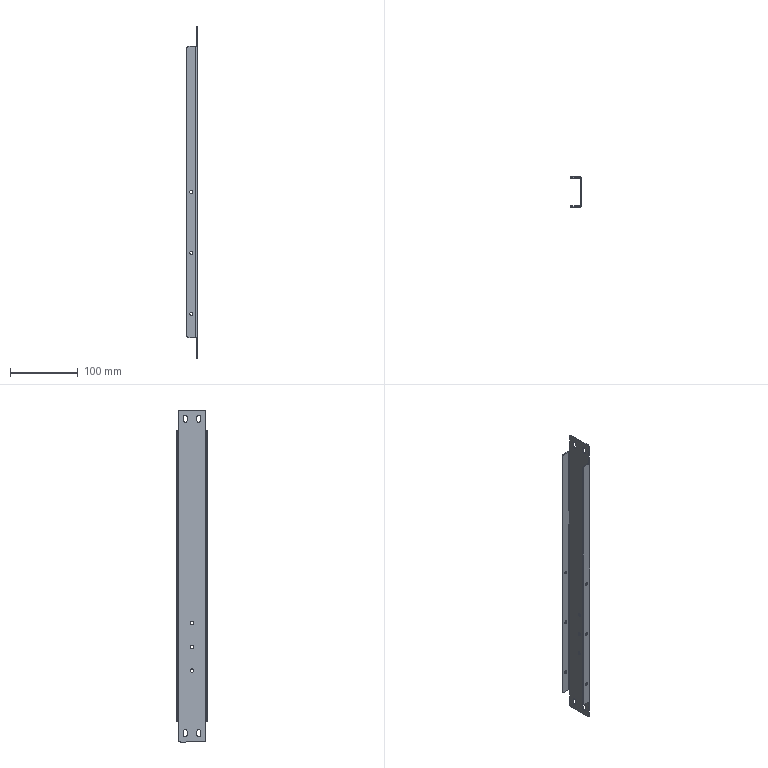Component | SolidWorks | MoldedCaseMountingBeamTwo100-7 | 1 solid | 72 faces | volume 48368 mm3 | cylinder 42 | plane 30 | commonest cylinder face diameters 4.5 x12 5.5 x12 6 x8 5 x6 4.473 x2 1.473 x2